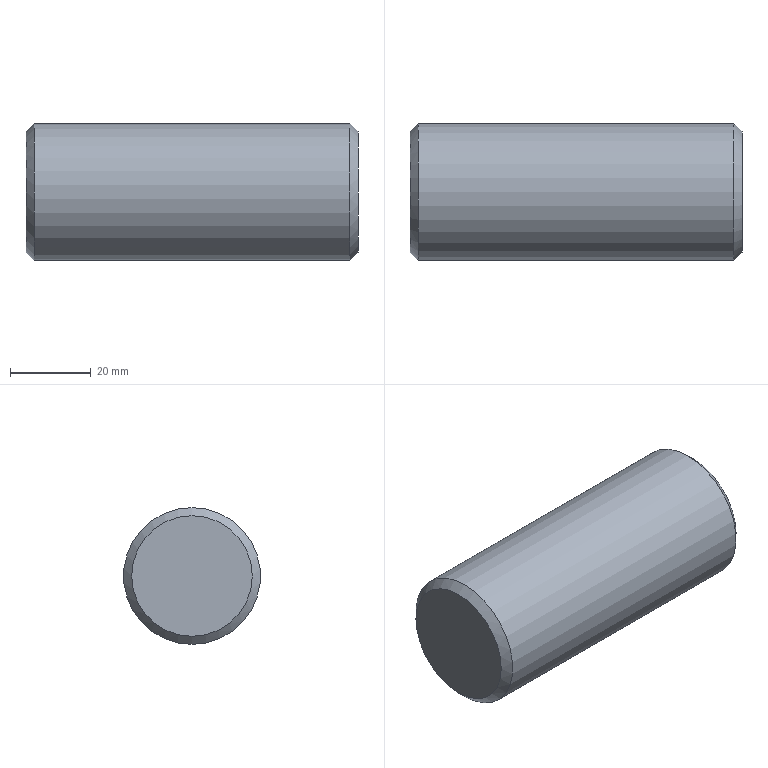Component | NX | 6_PISTON_PIN_3 | 1 solid | 5 faces | box 82 x 33.8 x 33.8 mm | volume 73168 mm3 | plane 2 | cone 2 | cylinder 1 | commonest cylinder face diameters 33.8 x1
STEP:
#1=CARTESIAN_POINT('',(0.,0.,0.));
#2=DIRECTION('',(0.,0.,1.));
#3=DIRECTION('',(1.,0.,0.));
#4=AXIS2_PLACEMENT_3D('',#1,#2,#3);
#5=CARTESIAN_POINT('',(-472.,226.604,-16.9));
#6=VERTEX_POINT('',#5);
#7=CARTESIAN_POINT('',(-472.,226.604,0.));
#8=DIRECTION('',(1.,0.,0.));
#9=DIRECTION('',(0.,0.,-1.));
#10=AXIS2_PLACEMENT_3D('',#7,#8,#9);
#11=CIRCLE('',#10,16.9);
#12=CARTESIAN_POINT('',(-392.,226.604,0.));
#13=DIRECTION('',(-1.,0.,0.));
#14=DIRECTION('',(0.,0.,1.));
#15=AXIS2_PLACEMENT_3D('',#12,#13,#14);
#16=CYLINDRICAL_SURFACE('',#15,16.9);
#17=CARTESIAN_POINT('',(9.425,80.));
#18=DIRECTION('',(-1.,0.));
#19=VECTOR('',#18,1.);
#20=LINE('',#17,#19);
#21=(GEOMETRIC_REPRESENTATION_CONTEXT(2)PARAMETRIC_REPRESENTATION_CONTEXT()REPRESENTATION_CONTEXT('',''));
#22=DEFINITIONAL_REPRESENTATION('',(#20),#21);
#23=PCURVE('',#16,#22);
#24=CARTESIAN_POINT('',(-472.,226.604,0.));
#25=DIRECTION('',(1.,0.,0.));
#26=DIRECTION('',(0.,0.,-1.));
#27=AXIS2_PLACEMENT_3D('',#24,#25,#26);
#28=CONICAL_SURFACE('',#27,16.9,0.7854);
#29=CARTESIAN_POINT('',(0.,0.));
#30=DIRECTION('',(1.,0.));
#31=VECTOR('',#30,1.);
#32=LINE('',#29,#31);
#33=(GEOMETRIC_REPRESENTATION_CONTEXT(2)PARAMETRIC_REPRESENTATION_CONTEXT()REPRESENTATION_CONTEXT('',''));
#34=DEFINITIONAL_REPRESENTATION('',(#32),#33);
#35=PCURVE('',#28,#34);
#36=SURFACE_CURVE('',#11,(#23,#35),.PCURVE_S1.);
#37=EDGE_CURVE('',#6,#6,#36,.T.);
#38=ORIENTED_EDGE('',*,*,#37,.T.);
#39=CARTESIAN_POINT('',(-394.,226.604,-16.9));
#40=VERTEX_POINT('',#39);
#41=CARTESIAN_POINT('',(-394.,226.604,-16.9));
#42=CARTESIAN_POINT('',(-472.,226.604,-16.9));
#43=B_SPLINE_CURVE_WITH_KNOTS('',1,(#41,#42),.UNSPECIFIED.,.F.,.F.,(2,2),(2.,80.),.PIECEWISE_BEZIER_KNOTS.);
#44=CARTESIAN_POINT('',(3.142,0.));
#45=DIRECTION('',(0.,1.));
#46=VECTOR('',#45,1.);
#47=LINE('',#44,#46);
#48=(GEOMETRIC_REPRESENTATION_CONTEXT(2)PARAMETRIC_REPRESENTATION_CONTEXT()REPRESENTATION_CONTEXT('',''));
#49=DEFINITIONAL_REPRESENTATION('',(#47),#48);
#50=PCURVE('',#16,#49);
#51=CARTESIAN_POINT('',(9.425,0.));
#52=DIRECTION('',(0.,1.));
#53=VECTOR('',#52,1.);
#54=LINE('',#51,#53);
#55=(GEOMETRIC_REPRESENTATION_CONTEXT(2)PARAMETRIC_REPRESENTATION_CONTEXT()REPRESENTATION_CONTEXT('',''));
#56=DEFINITIONAL_REPRESENTATION('',(#54),#55);
#57=PCURVE('',#16,#56);
#58=SEAM_CURVE('',#43,(#50,#57),.PCURVE_S1.);
#59=EDGE_CURVE('',#40,#6,#58,.T.);
#60=ORIENTED_EDGE('',*,*,#59,.F.);
#61=CARTESIAN_POINT('',(-394.,226.604,0.));
#62=DIRECTION('',(-1.,0.,0.));
#63=DIRECTION('',(0.,0.,-1.));
#64=AXIS2_PLACEMENT_3D('',#61,#62,#63);
#65=CIRCLE('',#64,16.9);
#66=CARTESIAN_POINT('',(3.142,2.));
#67=DIRECTION('',(1.,0.));
#68=VECTOR('',#67,1.);
#69=LINE('',#66,#68);
#70=(GEOMETRIC_REPRESENTATION_CONTEXT(2)PARAMETRIC_REPRESENTATION_CONTEXT()REPRESENTATION_CONTEXT('',''));
#71=DEFINITIONAL_REPRESENTATION('',(#69),#70);
#72=PCURVE('',#16,#71);
#73=CARTESIAN_POINT('',(-392.,226.604,0.));
#74=DIRECTION('',(-1.,0.,0.));
#75=DIRECTION('',(0.,0.,1.));
#76=AXIS2_PLACEMENT_3D('',#73,#74,#75);
#77=CONICAL_SURFACE('',#76,14.9,0.7854);
#78=CARTESIAN_POINT('',(3.142,2.));
#79=DIRECTION('',(1.,0.));
#80=VECTOR('',#79,1.);
#81=LINE('',#78,#80);
#82=(GEOMETRIC_REPRESENTATION_CONTEXT(2)PARAMETRIC_REPRESENTATION_CONTEXT()REPRESENTATION_CONTEXT('',''));
#83=DEFINITIONAL_REPRESENTATION('',(#81),#82);
#84=PCURVE('',#77,#83);
#85=SURFACE_CURVE('',#65,(#72,#84),.PCURVE_S1.);
#86=EDGE_CURVE('',#40,#40,#85,.T.);
#87=ORIENTED_EDGE('',*,*,#86,.T.);
#88=ORIENTED_EDGE('',*,*,#59,.T.);
#89=EDGE_LOOP('',(#38,#60,#87,#88));
#90=FACE_BOUND('',#89,.T.);
#91=ADVANCED_FACE('',(#90),#16,.T.);
#92=CARTESIAN_POINT('',(-392.,226.604,-14.9));
#93=VERTEX_POINT('',#92);
#94=CARTESIAN_POINT('',(-392.,226.604,0.));
#95=DIRECTION('',(1.,0.,0.));
#96=DIRECTION('',(0.,0.,-1.));
#97=AXIS2_PLACEMENT_3D('',#94,#95,#96);
#98=CIRCLE('',#97,14.9);
#99=CARTESIAN_POINT('',(-392.,226.604,0.));
#100=DIRECTION('',(1.,0.,0.));
#101=DIRECTION('',(0.,0.,-1.));
#102=AXIS2_PLACEMENT_3D('',#99,#100,#101);
#103=PLANE('',#102);
#104=CARTESIAN_POINT('',(0.,0.));
#105=DIRECTION('',(1.,0.));
#106=AXIS2_PLACEMENT_2D('',#104,#105);
#107=CIRCLE('',#106,14.9);
#108=(GEOMETRIC_REPRESENTATION_CONTEXT(2)PARAMETRIC_REPRESENTATION_CONTEXT()REPRESENTATION_CONTEXT('',''));
#109=DEFINITIONAL_REPRESENTATION('',(#107),#108);
#110=PCURVE('',#103,#109);
#111=CARTESIAN_POINT('',(9.425,0.));
#112=DIRECTION('',(-1.,0.));
#113=VECTOR('',#112,1.);
#114=LINE('',#111,#113);
#115=(GEOMETRIC_REPRESENTATION_CONTEXT(2)PARAMETRIC_REPRESENTATION_CONTEXT()REPRESENTATION_CONTEXT('',''));
#116=DEFINITIONAL_REPRESENTATION('',(#114),#115);
#117=PCURVE('',#77,#116);
#118=SURFACE_CURVE('',#98,(#110,#117),.PCURVE_S1.);
#119=EDGE_CURVE('',#93,#93,#118,.T.);
#120=ORIENTED_EDGE('',*,*,#119,.T.);
#121=EDGE_LOOP('',(#120));
#122=FACE_BOUND('',#121,.T.);
#123=ADVANCED_FACE('',(#122),#103,.T.);
#124=CARTESIAN_POINT('',(-474.,226.604,-14.9));
#125=VERTEX_POINT('',#124);
#126=CARTESIAN_POINT('',(-474.,226.604,0.));
#127=DIRECTION('',(-1.,0.,0.));
#128=DIRECTION('',(0.,0.,-1.));
#129=AXIS2_PLACEMENT_3D('',#126,#127,#128);
#130=CIRCLE('',#129,14.9);
#131=CARTESIAN_POINT('',(-474.,226.604,0.));
#132=DIRECTION('',(1.,0.,0.));
#133=DIRECTION('',(0.,0.,-1.));
#134=AXIS2_PLACEMENT_3D('',#131,#132,#133);
#135=PLANE('',#134);
#136=CARTESIAN_POINT('',(14.9,0.));
#137=CARTESIAN_POINT('',(14.9,-25.808));
#138=CARTESIAN_POINT('',(-7.45,-12.904));
#139=CARTESIAN_POINT('',(-29.8,-0.));
#140=CARTESIAN_POINT('',(-7.45,12.904));
#141=CARTESIAN_POINT('',(14.9,25.808));
#142=CARTESIAN_POINT('',(14.9,0.));
#143=(BOUNDED_CURVE()B_SPLINE_CURVE(2,(#136,#137,#138,#139,#140,#141,#142),.UNSPECIFIED.,.T.,.F.)B_SPLINE_CURVE_WITH_KNOTS((1,2,2,2,2,1),(-2.094,0.,2.094,4.189,6.283,8.378),.UNSPECIFIED.)CURVE()GEOMETRIC_REPRESENTATION_ITEM()RATIONAL_B_SPLINE_CURVE((1.,0.5,1.,0.5,1.,0.5,1.))REPRESENTATION_ITEM(''));
#144=(GEOMETRIC_REPRESENTATION_CONTEXT(2)PARAMETRIC_REPRESENTATION_CONTEXT()REPRESENTATION_CONTEXT('',''));
#145=DEFINITIONAL_REPRESENTATION('',(#143),#144);
#146=PCURVE('',#135,#145);
#147=CARTESIAN_POINT('',(6.283,-2.));
#148=DIRECTION('',(-1.,0.));
#149=VECTOR('',#148,1.);
#150=LINE('',#147,#149);
#151=(GEOMETRIC_REPRESENTATION_CONTEXT(2)PARAMETRIC_REPRESENTATION_CONTEXT()REPRESENTATION_CONTEXT('',''));
#152=DEFINITIONAL_REPRESENTATION('',(#150),#151);
#153=PCURVE('',#28,#152);
#154=SURFACE_CURVE('',#130,(#146,#153),.PCURVE_S1.);
#155=EDGE_CURVE('',#125,#125,#154,.T.);
#156=ORIENTED_EDGE('',*,*,#155,.T.);
#157=EDGE_LOOP('',(#156));
#158=FACE_BOUND('',#157,.T.);
#159=ADVANCED_FACE('',(#158),#135,.F.);
#160=ORIENTED_EDGE('',*,*,#155,.F.);
#161=CARTESIAN_POINT('',(-474.,226.604,-14.9));
#162=CARTESIAN_POINT('',(-472.,226.604,-16.9));
#163=B_SPLINE_CURVE_WITH_KNOTS('',1,(#161,#162),.UNSPECIFIED.,.F.,.F.,(2,2),(-2.828,0.),.PIECEWISE_BEZIER_KNOTS.);
#164=CARTESIAN_POINT('',(6.283,0.));
#165=DIRECTION('',(0.,1.));
#166=VECTOR('',#165,1.);
#167=LINE('',#164,#166);
#168=(GEOMETRIC_REPRESENTATION_CONTEXT(2)PARAMETRIC_REPRESENTATION_CONTEXT()REPRESENTATION_CONTEXT('',''));
#169=DEFINITIONAL_REPRESENTATION('',(#167),#168);
#170=PCURVE('',#28,#169);
#171=CARTESIAN_POINT('',(0.,0.));
#172=DIRECTION('',(0.,1.));
#173=VECTOR('',#172,1.);
#174=LINE('',#171,#173);
#175=(GEOMETRIC_REPRESENTATION_CONTEXT(2)PARAMETRIC_REPRESENTATION_CONTEXT()REPRESENTATION_CONTEXT('',''));
#176=DEFINITIONAL_REPRESENTATION('',(#174),#175);
#177=PCURVE('',#28,#176);
#178=SEAM_CURVE('',#163,(#170,#177),.PCURVE_S1.);
#179=EDGE_CURVE('',#125,#6,#178,.T.);
#180=ORIENTED_EDGE('',*,*,#179,.T.);
#181=ORIENTED_EDGE('',*,*,#37,.F.);
#182=ORIENTED_EDGE('',*,*,#179,.F.);
#183=EDGE_LOOP('',(#160,#180,#181,#182));
#184=FACE_BOUND('',#183,.T.);
#185=ADVANCED_FACE('',(#184),#28,.T.);
#186=ORIENTED_EDGE('',*,*,#86,.F.);
#187=CARTESIAN_POINT('',(-392.,226.604,-14.9));
#188=CARTESIAN_POINT('',(-394.,226.604,-16.9));
#189=B_SPLINE_CURVE_WITH_KNOTS('',1,(#187,#188),.UNSPECIFIED.,.F.,.F.,(2,2),(0.,2.828),.PIECEWISE_BEZIER_KNOTS.);
#190=CARTESIAN_POINT('',(3.142,0.));
#191=DIRECTION('',(0.,1.));
#192=VECTOR('',#191,1.);
#193=LINE('',#190,#192);
#194=(GEOMETRIC_REPRESENTATION_CONTEXT(2)PARAMETRIC_REPRESENTATION_CONTEXT()REPRESENTATION_CONTEXT('',''));
#195=DEFINITIONAL_REPRESENTATION('',(#193),#194);
#196=PCURVE('',#77,#195);
#197=CARTESIAN_POINT('',(9.425,0.));
#198=DIRECTION('',(0.,1.));
#199=VECTOR('',#198,1.);
#200=LINE('',#197,#199);
#201=(GEOMETRIC_REPRESENTATION_CONTEXT(2)PARAMETRIC_REPRESENTATION_CONTEXT()REPRESENTATION_CONTEXT('',''));
#202=DEFINITIONAL_REPRESENTATION('',(#200),#201);
#203=PCURVE('',#77,#202);
#204=SEAM_CURVE('',#189,(#196,#203),.PCURVE_S1.);
#205=EDGE_CURVE('',#93,#40,#204,.T.);
#206=ORIENTED_EDGE('',*,*,#205,.F.);
#207=ORIENTED_EDGE('',*,*,#119,.F.);
#208=ORIENTED_EDGE('',*,*,#205,.T.);
#209=EDGE_LOOP('',(#186,#206,#207,#208));
#210=FACE_BOUND('',#209,.T.);
#211=ADVANCED_FACE('',(#210),#77,.T.);
#212=CLOSED_SHELL('',(#91,#123,#159,#185,#211));
#213=MANIFOLD_SOLID_BREP('',#212);
#214=(LENGTH_UNIT()NAMED_UNIT(*)SI_UNIT(.MILLI.,.METRE.));
#215=UNCERTAINTY_MEASURE_WITH_UNIT(LENGTH_MEASURE(0.00001),#214,'','');
#216=(NAMED_UNIT(*)PLANE_ANGLE_UNIT()SI_UNIT($,.RADIAN.));
#217=(NAMED_UNIT(*)SI_UNIT($,.STERADIAN.)SOLID_ANGLE_UNIT());
#218=(GEOMETRIC_REPRESENTATION_CONTEXT(3)GLOBAL_UNCERTAINTY_ASSIGNED_CONTEXT((#215))GLOBAL_UNIT_ASSIGNED_CONTEXT((#214,#216,#217))REPRESENTATION_CONTEXT('',''));
#219=ADVANCED_BREP_SHAPE_REPRESENTATION('',(#4,#213),#218);